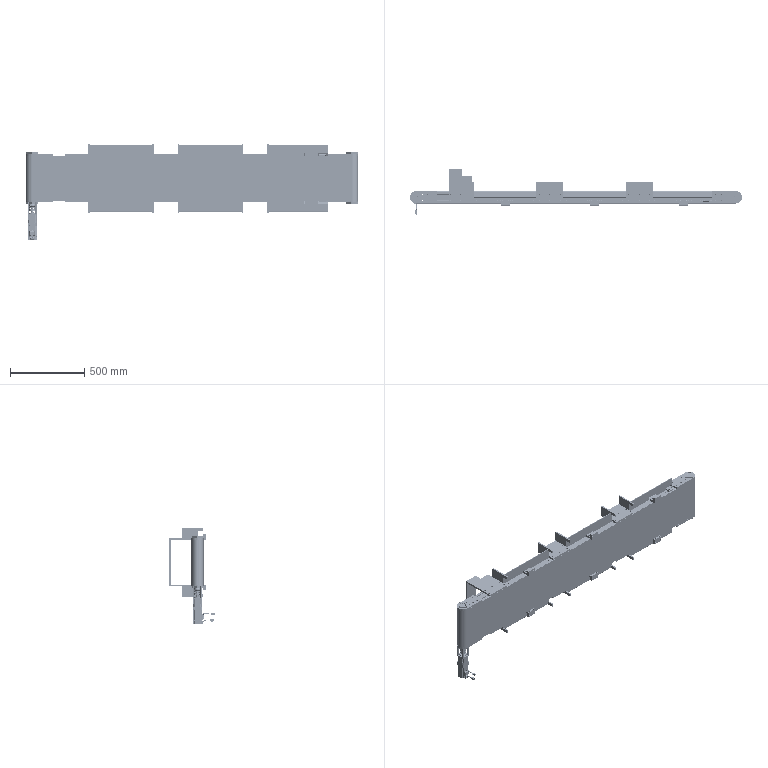Assembly | SolidWorks | mm | 172 component files | 363 solids | 12033 faces | box 2231 x 303.69 x 644.5 mm | volume 22318651 mm3 | plane 6929 | cylinder 3291 | cone 1285 | torus 238 | sphere 160 | spline 130 | commonest cylinder face diameters 8 x392 11 x192 6.6 x192 6 x169 9 x160 13 x160 1 x141 2 x135
Bill of materials:
Q1-A12-S21-Q1A-01A | 2 | S-45C | Flat plate with one rounded end. The rounded end has a large central bore with a ring of small holes around it. The rectangular section has two rows of three holes and two parallel slots on top, and there are notches along the side edges.
Q1-A12-S21-Q1A-02A | 2 | Q235-Steel | Long rectangular bar with two through holes along its length, and chamfers on the two lower long edges.
Q1-A12-S21-Q1A-03A | 1 | SUJ2 | Cylindrical body made of two coaxial larger-diameter sections separated by a narrower neck, with small stepped shaft stubs at both ends.
Q1-CPDW40-16-16 | 1 |  | Cylindrical shaft coupling with two split clamp hubs at the ends and a central spacer ring, joined by thin disc layers held by axial pins or bolts.
Q1-HNTA8-6 | 36 |  | Small block with a trapezoidal top section over a narrower rectangular bottom tongue, giving a stepped profile. It has a single through hole with a chamfered or countersunk entry.
Q1-PAB060-10-S2-P2-14-50-70-Q4 | 1 |  | Square-flanged housing with a round pilot boss and an output shaft on top. Its long body has square edges and longitudinal grooves, and a square base section has a side hole.
Q1-QSQF042L1U2 | 1 |  | Square-flanged, elongated body with a front shaft and a pilot boss. Two side-mounted connector housings have short bent cable leads that end in multi-pin rectangular connector plugs.
Q1-VAFD10-75-F10-Q6-N5 | 4 |  | Long cylindrical pin that steps down at one end to a short smaller-diameter head, with a narrow neck or groove between the head and the main body.
Q1-GNFS8-4080-220 | 6 | 6061 | Extruded profile segment with a rectangular cross-section, roughly 1 x 2 in proportion. It has slots on all sides, a central hollow core and two circular core holes, and a rectangular notch cut partway along the length on both narrow sides.
Q1-HBKTS8-C-SEP | 40 | 6061 | L-shaped angle bracket with a diagonal gusset rib. Each leg carries a socket-head screw that passes through it to a wedge-shaped slot-nut-like piece on the outer face.
Q1-A12-S21-Q1C-01B | 2 | S-45C | Flat plate with one rounded end. The rounded end has a large bore with 4 small holes around it, and the rectangular section has 7 larger holes. Small cross holes or notches appear on one side edge.
Q1-A12-S21-Q1C-02A | 1 | SUJ2 | Cylindrical body made of two coaxial large-diameter sections separated by a narrow neck, with short small-diameter shaft stubs and shoulders at both ends.
Q1-A12-S21-Q1C-03A | 1 | Q235-Steel | Long, slender rectangular bar or thick strip with two small holes drilled into one narrow end face.
Q1-A12-S21-Q1D-01A | 2 | Q235-Steel | Rectangular block with four counterbored through holes in a rectangular pattern, chamfers along two opposite top edges, two raised pads or rails on the underside, and one blind hole in a side face.
Q1-A12-S21-Q4-01A | 4 | SUS-304 | Thin rectangular sheet panel with a joggled (offset) band running across its full width and four small holes near the corners.
Q1-A12-S21-Q4-02A | 6 | SUS-304 | Thin rectangular sheet panel with a joggled offset band across its width and four small corner holes. It looks like the previous panel but is proportionally longer.
Q1-A12-S21-Q4-03A | 4 | White Plastic Steel POM | Thick rectangular plate with six counterbored holes in a 2x3 grid near one edge, three small holes in that edge face, and two short projections on the underside at that edge.
Q1-A12-S21-Q4-05B | 4 | SUS-304 | Bent sheet profile: a horizontal flange with holes, a vertical web, and a hairpin bend at the top that turns into a long angled leg. The flange is split into two tabs by a central notch.
Q1-A12-S21-Q4-06B | 5 | White Plastic Steel POM | Flat L-shaped plate: a rectangular body with a narrow arm sticking out sideways from one top edge, and two small holes near the bottom edge of the body.
Q1-A12-S21-Q4-07B | 1 | SUS-304 | Bent sheet profile with a base flange, a vertical web, a hairpin top bend and an angled leg. The flange is split into one long and one short tab with holes, and the web has rectangular notches in its lower edge between and beyond the tabs.
Q1-A12-S21-Q4-08B | 1 | SUS-304 | Bent sheet profile that looks the same as unnamed part but is shown inverted: a flange with one long and one short tab with holes, a web, a hairpin bend and an angled leg.
Q1-A12-S21-Q4-09B | 5 | White Plastic Steel POM | Flat L-shaped plate with a narrow arm sticking out sideways along one edge and two small holes near the opposite edge. It looks like unnamed part turned over or rotated.
Q1-A12-S21-Q4-10A | 1 | White Plastic Steel POM | Thick plate with a rectangular notch cut from one corner, six counterbored holes in a 2x3 grid near the opposite edge, three small holes in one edge face, and two short projections on the underside.
Q1-A12-S21-Q4-11A | 1 | White Plastic Steel POM | Thick plate with a rectangular notch cut from one corner and six holes in a 2x3 grid. Two narrow raised strips run across the full length of the face shown, and there are three small holes in one edge face. It looks like unnamed part seen from its other side.
Q1-A12-S21-Q4-12A | 1 | White Plastic Steel POM | Thin flat rectangular plate, elongated, with six small through holes: a row of three near each short end.
Q1-A12-S21-Q1E-02A | 6 | Q235-Steel | Rectangular block with two round through holes in its largest face and one chamfer along a single long edge.
Q1-A12-S21-Q4E-01A | 6 | Q235-Steel | Stepped rectangular block: a higher section with two larger through holes, a lower ledge with two smaller through holes, and a narrow rib sticking out of the underside.
Q1-GNFS8-4080-2030 | 2 | 6061 | Long straight extruded bar with a constant slotted cross-section: a rectangle about 2:1 with rounded outer corners, T-shaped slots on all faces, two round core bores, and a central hollow.
Q1-HBLTDS300-4.55 | 1 |  | Long flat bar with fully rounded (semicircular) ends, giving a stadium/obround outline, and a uniform rectangular section through its height.
Mates:
1. coincident | Q1-A12-S21-Q1A.SLDASQ-1/Q1-A12-S21-Q1A-01A-2 face at (48.5, 0, 162.5) dir (0, 0, 1) | Q1-A12-S21-Q1C.SLDASQ-1/Q1-A12-S21-Q1C-01B-1 face at (2089.5, 0, 162.5) dir (0, 0, 1)
2. coincident | Q1-A12-S21-Q1A.SLDASQ-1/Q1-A12-S21-Q1A-01A-2 face at (-41.5, 41.5, 162.5) dir (0, 1, 0) | Q1-A12-S21-Q1C.SLDASQ-1/Q1-A12-S21-Q1C-01B-1 face at (2189.5, 41.5, 162.5) dir (0, 1, 0)
3. distance | Q1-A12-S21-Q1C.SLDASQ-1 plane at (2148, 0, 147.5) dir (-1, 0, 0) | Q1-A12-S21-Q1A.SLDASQ-1 plane at (0, 0, -147.5) dir (1, 0, 0)
4. coincident | Q1-A12-S21-Q1A.SLDASQ-1 plane at (48.5, 0, 0) dir (0, 0, 1) | Q1-HBLTDS300-4.55-1 plane at (0, 0, 0) dir (0, 0, 1)
5. concentric | Q1-A12-S21-Q1A.SLDASQ-1/Q1-A12-S21-Q1A-03A-1 face at (0, 0, -250) dir (0, 0, -1) r 40 | Q1-HBLTDS300-4.55-1 face at (0, 0, -5) dir (0, 0, -1) r 40
6. parallel | Q1-A12-S21-Q1C.SLDASQ-1/Q1-A12-S21-Q1C-01B-1 face at (2189.5, 41.5, 162.5) dir (0, 1, 0) | Q1-HBLTDS300-4.55-1 face at (2148, 41.4, -150) dir (0, 1, 0)
7. coincident | Q1-A12-S21-Q1A.SLDASQ-1/Q1-A12-S21-Q1A-01A-2 face at (-41.5, 41.5, 150) dir (0, 0, -1) | Q1-GNFS8-4080-2030-1 face at (2078.5, 15, 150) dir (0, 0, 1)
8. width | Q1-GNFS8-4080-2030-1 face at (2078.5, 40, 135) dir (0, 1, 0) | Q1-GNFS8-4080-2030-1 face at (2078.5, -40, 147) dir (0, -1, 0) | Q1-A12-S21-Q1A.SLDASQ-1/Q1-A12-S21-Q1A-01A-2 face at (-41.5, -41.5, 162.5) dir (0, -1, 0) | Q1-A12-S21-Q1A.SLDASQ-1/Q1-A12-S21-Q1A-01A-2 face at (-41.5, 41.5, 162.5) dir (0, 1, 0)
9. coincident | Q1-A12-S21-Q1A.SLDASQ-1/Q1-A12-S21-Q1A-02A-2 face at (48.5, -35, 152.5) dir (1, 0, 0) | Q1-GNFS8-4080-2030-1 face at (48.5, 37, 113) dir (-1, 0, 0)
10. coincident | Q1-GNFS8-4080-2030-1 face at (2078.5, 40, 113) dir (0, 1, 0) | Q1-GNFS8-4080-2030-2 face at (2078.5, 40, -147) dir (0, 1, 0)
11. coincident | Q1-A12-S21-Q1A.SLDASQ-1/Q1-A12-S21-Q1A-01A-1 face at (-41.5, -15, -150) dir (0, 0, 1) | Q1-GNFS8-4080-2030-2 face at (2078.5, -15, -150) dir (0, 0, -1)
12. coincident | Q1-A12-S21-Q1A.SLDASQ-1/Q1-A12-S21-Q1A-02A-1 face at (48.5, 35, -152.5) dir (1, 0, 0) | Q1-GNFS8-4080-2030-2 face at (48.5, 37, -147) dir (-1, 0, 0)
13. coincident | Q1-GNFS8-4080-2030-2 face at (2078.5, 40, -125) dir (0, 1, 0) | Q1-GNFS8-4080-220-1 face at (73.5, 40, -110) dir (0, 1, 0)
14. coincident | Q1-GNFS8-4080-2030-2 face at (48.5, 37, -147) dir (-1, 0, 0) | Q1-GNFS8-4080-220-1 face at (48.5, 25, -110) dir (-1, 0, 0)
15. coincident | Q1-GNFS8-4080-2030-2 face at (2078.5, 37, -110) dir (0, 0, 1) | Q1-GNFS8-4080-220-1 face at (51.5, 37, -110) dir (0, 0, -1)
16. coincident | Q1-GNFS8-4080-220-1 face at (73.5, 40, -110) dir (0, 1, 0) | Q1-GNFS8-4080-220-2 face at (2063.5, 40, -110) dir (0, 1, 0)
17. coincident | Q1-GNFS8-4080-2030-1 face at (2078.5, -15, 110) dir (0, 0, -1) | Q1-GNFS8-4080-220-2 face at (2041.5, 37, 110) dir (0, 0, 1)
18. coincident | Q1-GNFS8-4080-2030-2 face at (2078.5, 37, -147) dir (1, 0, 0) | Q1-GNFS8-4080-220-2 face at (2078.5, 15, -110) dir (1, 0, 0)
19. width | Q1-HBKTS8-C-SEP-1 face at (2038.5, 35, -110) dir (0, 1, 0) | Q1-HBKTS8-C-SEP-1 face at (2038.5, 5, -110) dir (0, -1, 0) | Q1-GNFS8-4080-220-2 face at (2038.5, 15, -110) dir (0, 1, 0) | Q1-GNFS8-4080-220-2 face at (2044, 25, -110) dir (0, -1, 0)
20. coincident | Q1-GNFS8-4080-220-2 face at (2038.5, 25, -110) dir (-1, 0, 0) | Q1-HBKTS8-C-SEP-1 face at (2038.5, 35, -59) dir (1, 0, 0)
21. coincident | Q1-GNFS8-4080-2030-2 face at (2078.5, 37, -110) dir (0, 0, 1) | Q1-HBKTS8-C-SEP-1 face at (2038.5, 35, -110) dir (0, 0, -1)
22. width | Q1-HBKTS8-C-SEP-2 face at (2038.5, -5, -110) dir (0, 1, 0) | Q1-HBKTS8-C-SEP-2 face at (2038.5, -35, -110) dir (0, -1, 0) | Q1-GNFS8-4080-220-2 face at (2044, -15, -110) dir (0, -1, 0) | Q1-GNFS8-4080-220-2 face at (2038.5, -25, -110) dir (0, 1, 0)
23. coincident | Q1-GNFS8-4080-220-2 face at (2038.5, -15, -110) dir (-1, 0, 0) | Q1-HBKTS8-C-SEP-2 face at (2038.5, -5, -59) dir (1, 0, 0)
24. coincident | Q1-GNFS8-4080-2030-2 face at (2078.5, 15, -110) dir (0, 0, 1) | Q1-HBKTS8-C-SEP-2 face at (2038.5, -5, -110) dir (0, 0, -1)
25. coincident | Q1-HBKTS8-C-SEP-1 face at (2038.5, 35, -110) dir (0, 1, 0) | Q1-HBKTS8-C-SEP-3 face at (2038.5, 35, 110) dir (0, 1, 0)
26. coincident | Q1-HBKTS8-C-SEP-1 face at (2029.5, 35, -81) dir (-1, 0, 0) | Q1-HBKTS8-C-SEP-3 face at (2029.5, 35, 59) dir (-1, 0, 0)
27. coincident | Q1-GNFS8-4080-2030-1 face at (2078.5, -15, 110) dir (0, 0, -1) | Q1-HBKTS8-C-SEP-3 face at (1987.5, 35, 110) dir (0, 0, 1)
28. coincident | Q1-HBKTS8-C-SEP-2 face at (2038.5, -5, -110) dir (0, 1, 0) | Q1-HBKTS8-C-SEP-4 face at (2038.5, -5, 110) dir (0, 1, 0)
29. coincident | Q1-HBKTS8-C-SEP-3 face at (2029.5, 35, 59) dir (-1, 0, 0) | Q1-HBKTS8-C-SEP-4 face at (2029.5, -5, 59) dir (-1, 0, 0)
30. coincident | Q1-HBKTS8-C-SEP-3 face at (2009.5, 35, 101) dir (0, 0, -1) | Q1-HBKTS8-C-SEP-4 face at (2009.5, -5, 101) dir (0, 0, -1)
31. coincident | Q1-HBKTS8-C-SEP-2 face at (2038.5, -5, -110) dir (0, 1, 0) | Q1-HBKTS8-C-SEP-5 face at (88.5, -5, -110) dir (0, 1, 0)
32. coincident | Q1-GNFS8-4080-2030-2 face at (2078.5, 15, -110) dir (0, 0, 1) | Q1-HBKTS8-C-SEP-5 face at (88.5, -35, -110) dir (0, 0, -1)
33. coincident | Q1-GNFS8-4080-220-1 face at (88.5, 15, -110) dir (1, 0, 0) | Q1-HBKTS8-C-SEP-5 face at (88.5, -35, -59) dir (-1, 0, 0)
34. coincident | Q1-HBKTS8-C-SEP-1 face at (2038.5, 35, -110) dir (0, 1, 0) | Q1-HBKTS8-C-SEP-6 face at (88.5, 35, -110) dir (0, 1, 0)
35. coincident | Q1-GNFS8-4080-2030-2 face at (2078.5, 37, -110) dir (0, 0, 1) | Q1-HBKTS8-C-SEP-6 face at (88.5, 5, -110) dir (0, 0, -1)
36. coincident | Q1-GNFS8-4080-220-1 face at (88.5, 37, -110) dir (1, 0, 0) | Q1-HBKTS8-C-SEP-6 face at (88.5, 5, -59) dir (-1, 0, 0)
37. coincident | Q1-HBKTS8-C-SEP-6 face at (88.5, 35, -110) dir (0, 1, 0) | Q1-HBKTS8-C-SEP-7 face at (88.5, 35, 110) dir (0, 1, 0)
38. coincident | Q1-HBKTS8-C-SEP-6 face at (97.5, 5, -81) dir (1, 0, 0) | Q1-HBKTS8-C-SEP-7 face at (97.5, 5, 59) dir (1, 0, 0)
39. coincident | Q1-GNFS8-4080-2030-1 face at (2078.5, 25, 110) dir (0, 0, -1) | Q1-HBKTS8-C-SEP-7 face at (139.5, 5, 110) dir (0, 0, 1)
40. coincident | Q1-HBKTS8-C-SEP-5 face at (88.5, -5, -110) dir (0, 1, 0) | Q1-HBKTS8-C-SEP-8 face at (88.5, -5, 110) dir (0, 1, 0)
41. coincident | Q1-HBKTS8-C-SEP-7 face at (97.5, 5, 59) dir (1, 0, 0) | Q1-HBKTS8-C-SEP-8 face at (97.5, -35, 59) dir (1, 0, 0)
42. coincident | Q1-HBKTS8-C-SEP-7 face at (117.5, 5, 101) dir (0, 0, -1) | Q1-HBKTS8-C-SEP-8 face at (117.5, -35, 101) dir (0, 0, -1)
43. coincident | Q1-GNFS8-4080-2030-2 face at (2078.5, 40, -125) dir (0, 1, 0) | Q1-A12-S21-Q1B.SLDASQ-1/Q1-GNFS8-4080-220-1 face at (1755.5, 40, 110) dir (0, 1, 0)
44. coincident | Q1-GNFS8-4080-2030-2 face at (2078.5, 37, -110) dir (0, 0, 1) | Q1-A12-S21-Q1B.SLDASQ-1/Q1-GNFS8-4080-220-1 face at (1755.5, 37, -110) dir (0, 0, -1)
45. coincident | Q1-A12-S21-Q1B.SLDASQ-1/Q1-GNFS8-4080-220-1 face at (1733.5, 40, 110) dir (0, 1, 0) | Q1-A12-S21-Q1B.SLDASQ-2/Q1-GNFS8-4080-220-1 face at (1305.5, 40, 110) dir (0, 1, 0)
46. coincident | Q1-GNFS8-4080-2030-2 face at (2078.5, 37, -110) dir (0, 0, 1) | Q1-A12-S21-Q1B.SLDASQ-2/Q1-GNFS8-4080-220-1 face at (1305.5, 37, -110) dir (0, 0, -1)
47. coincident | Q1-GNFS8-4080-2030-2 face at (2078.5, 40, -125) dir (0, 1, 0) | Q1-A12-S21-Q1B.SLDASQ-3/Q1-GNFS8-4080-220-1 face at (855.5, 40, 110) dir (0, 1, 0)
48. coincident | Q1-GNFS8-4080-2030-2 face at (2078.5, 37, -110) dir (0, 0, 1) | Q1-A12-S21-Q1B.SLDASQ-3/Q1-GNFS8-4080-220-1 face at (855.5, 37, -110) dir (0, 0, -1)
49. coincident | Q1-GNFS8-4080-2030-2 face at (2078.5, 40, -125) dir (0, 1, 0) | Q1-A12-S21-Q1B.SLDASQ-4/Q1-GNFS8-4080-220-1 face at (405.5, 40, 110) dir (0, 1, 0)
50. coincident | Q1-GNFS8-4080-2030-2 face at (2078.5, 15, -110) dir (0, 0, 1) | Q1-A12-S21-Q1B.SLDASQ-4/Q1-GNFS8-4080-220-1 face at (405.5, 37, -110) dir (0, 0, -1)
51. distance | Q1-GNFS8-4080-220-1 face at (48.5, 25, -110) dir (-1, 0, 0) | Q1-A12-S21-Q1B.SLDASQ-4/Q1-GNFS8-4080-220-1 face at (368.5, 37, 110) dir (-1, 0, 0)
52. distance | Q1-A12-S21-Q1B.SLDASQ-2/Q1-GNFS8-4080-220-1 face at (1268.5, 37, 110) dir (-1, 0, 0) | Q1-A12-S21-Q1B.SLDASQ-3/Q1-GNFS8-4080-220-1 face at (858.5, 25, 110) dir (1, 0, 0)
53. distance | Q1-A12-S21-Q1B.SLDASQ-1/Q1-GNFS8-4080-220-1 face at (1718.5, 37, 110) dir (-1, 0, 0) | Q1-A12-S21-Q1B.SLDASQ-2/Q1-GNFS8-4080-220-1 face at (1308.5, 25, 110) dir (1, 0, 0)
54. distance | Q1-A12-S21-Q1B.SLDASQ-3/Q1-GNFS8-4080-220-1 face at (818.5, 37, 110) dir (-1, 0, 0) | Q1-A12-S21-Q1B.SLDASQ-4/Q1-GNFS8-4080-220-1 face at (408.5, 25, 110) dir (1, 0, 0)
55. width | Q1-A12-S21-Q1D.SLDASQ-1/Q1-A12-S21-Q1D-01A-1 face at (1929.5, 30, 162.5) dir (0, 1, 0) | Q1-A12-S21-Q1D.SLDASQ-1/Q1-A12-S21-Q1D-01A-1 face at (1929.5, -30, 162.5) dir (0, -1, 0) | Q1-A12-S21-Q1C.SLDASQ-1/Q1-A12-S21-Q1C-01B-1 face at (2189.5, -41.5, 162.5) dir (0, -1, 0) | Q1-A12-S21-Q1C.SLDASQ-1/Q1-A12-S21-Q1C-01B-1 face at (2189.5, 41.5, 162.5) dir (0, 1, 0)
56. coincident | Q1-GNFS8-4080-2030-1 face at (2078.5, 37, 150) dir (0, 0, 1) | Q1-A12-S21-Q1D.SLDASQ-1/Q1-A12-S21-Q1D-01A-1 face at (1929.5, 30, 150) dir (0, 0, -1)
57. coincident | Q1-A12-S21-Q1C.SLDASQ-1/Q1-A12-S21-Q1C-01B-1 face at (1989.5, 41.5, 162.5) dir (-1, 0, 0) | Q1-A12-S21-Q1D.SLDASQ-1/Q1-RCB6-30-1 face at (1989.5, 0, 156.25) dir (1, 0, 0)
58. coincident | Q1-GNFS8-4080-2030-2 face at (2078.5, 25, -150) dir (0, 0, -1) | Q1-A12-S21-Q1D.SLDASQ-2/Q1-A12-S21-Q1D-01A-1 face at (1929.5, 30, -150) dir (0, 0, 1)
59. width | Q1-A12-S21-Q1C.SLDASQ-1/Q1-A12-S21-Q1C-01B-2 face at (2189.5, 41.5, -162.5) dir (0, 1, 0) | Q1-A12-S21-Q1C.SLDASQ-1/Q1-A12-S21-Q1C-01B-2 face at (2189.5, -41.5, -162.5) dir (0, -1, 0) | Q1-A12-S21-Q1D.SLDASQ-2/Q1-A12-S21-Q1D-01A-1 face at (1929.5, -30, -162.5) dir (0, -1, 0) | Q1-A12-S21-Q1D.SLDASQ-2/Q1-A12-S21-Q1D-01A-1 face at (1929.5, 30, -162.5) dir (0, 1, 0)
60. coincident | Q1-A12-S21-Q1C.SLDASQ-1/Q1-A12-S21-Q1C-01B-2 face at (1989.5, -41.5, -162.5) dir (-1, 0, 0) | Q1-A12-S21-Q1D.SLDASQ-2/Q1-RCB6-30-1 face at (1989.5, 0, -156.25) dir (1, 0, 0)
61. coincident | Q1-HBKTS8-C-SEP-3 face at (2038.5, 35, 110) dir (0, 1, 0) | Q1-A12-S21-Q4-01A-1 face at (1898.5, 35, -71.578) dir (0, -1, 0)
62. concentric | Q1-HBKTS8-C-SEP-1 face at (2026.5, 5, -98) dir (0, 1, 0) r 2.067 | Q1-A12-S21-Q4-01A-1 face at (2026.5, 39, -98) dir (0, 1, 0) r 2.75
63. parallel | Q1-GNFS8-4080-220-2 face at (2038.5, 25, -110) dir (-1, 0, 0) | Q1-A12-S21-Q4-01A-1 face at (2038.5, 39, 25.053) dir (1, 0, 0)
64. coincident | Q1-HBKTS8-C-SEP-7 face at (88.5, 35, 110) dir (0, 1, 0) | Q1-A12-S21-Q4-01A-2 face at (228.5, 35, -71.578) dir (0, -1, 0)
65. concentric | Q1-HBKTS8-C-SEP-6 face at (100.5, 35, -98) dir (0, -1, 0) r 2.067 | Q1-A12-S21-Q4-01A-2 face at (100.5, 39, -98) dir (0, 1, 0) r 2.75
66. parallel | Q1-GNFS8-4080-220-1 face at (88.5, 37, -110) dir (1, 0, 0) | Q1-A12-S21-Q4-01A-2 face at (88.5, 39, 110) dir (-1, 0, 0)
67. coincident | Q1-A12-S21-Q1B.SLDASQ-3/Q1-HBKTS8-C-SEP-7 face at (818.5, 35, -110) dir (0, 1, 0) | Q1-A12-S21-Q4-02A-1 face at (613.5, 35, -63) dir (0, -1, 0)
68. concentric | Q1-A12-S21-Q1B.SLDASQ-3/Q1-HBKTS8-C-SEP-7 face at (806.5, 5, -98) dir (0, 1, 0) r 2.067 | Q1-A12-S21-Q4-02A-1 face at (806.5, 39, -98) dir (0, 1, 0) r 2.75
69. parallel | Q1-A12-S21-Q1B.SLDASQ-3/Q1-GNFS8-4080-220-1 face at (818.5, 37, 110) dir (-1, 0, 0) | Q1-A12-S21-Q4-02A-1 face at (818.5, 39, 25.053) dir (1, 0, 0)
70. coincident | Q1-A12-S21-Q1B.SLDASQ-2/Q1-HBKTS8-C-SEP-7 face at (1268.5, 35, -110) dir (0, 1, 0) | Q1-A12-S21-Q4-02A-2 face at (1063.5, 35, -63) dir (0, -1, 0)
71. concentric | Q1-A12-S21-Q1B.SLDASQ-2/Q1-HBKTS8-C-SEP-7 face at (1256.5, 5, -98) dir (0, 1, 0) r 2.067 | Q1-A12-S21-Q4-02A-2 face at (1256.5, 39, -98) dir (0, 1, 0) r 2.75
72. parallel | Q1-A12-S21-Q1B.SLDASQ-2/Q1-GNFS8-4080-220-1 face at (1268.5, 37, 110) dir (-1, 0, 0) | Q1-A12-S21-Q4-02A-2 face at (1268.5, 39, 25.053) dir (1, 0, 0)
73. coincident | Q1-A12-S21-Q1B.SLDASQ-1/Q1-HBKTS8-C-SEP-7 face at (1718.5, 35, -110) dir (0, 1, 0) | Q1-A12-S21-Q4-02A-3 face at (1513.5, 35, -63) dir (0, -1, 0)
74. concentric | Q1-A12-S21-Q1B.SLDASQ-1/Q1-HBKTS8-C-SEP-7 face at (1706.5, 5, -98) dir (0, 1, 0) r 2.067 | Q1-A12-S21-Q4-02A-3 face at (1706.5, 39, -98) dir (0, 1, 0) r 2.75
75. parallel | Q1-A12-S21-Q1B.SLDASQ-1/Q1-GNFS8-4080-220-1 face at (1718.5, 37, 110) dir (-1, 0, 0) | Q1-A12-S21-Q4-02A-3 face at (1718.5, 39, 25.053) dir (1, 0, 0)
76. coincident | Q1-HBKTS8-C-SEP-4 face at (2038.5, -35, 110) dir (0, -1, 0) | Q1-A12-S21-Q4-01A-3 face at (1898.5, -35, 63) dir (0, 1, 0)
77. concentric | Q1-HBKTS8-C-SEP-4 face at (2026.5, -35, 98) dir (0, 1, 0) r 2.067 | Q1-A12-S21-Q4-01A-3 face at (2026.5, -39, 98) dir (0, -1, 0) r 2.75
78. parallel | Q1-GNFS8-4080-220-2 face at (2038.5, -37, -110) dir (-1, 0, 0) | Q1-A12-S21-Q4-01A-3 face at (2038.5, -35, 16) dir (1, 0, 0)
79. coincident | Q1-A12-S21-Q1B.SLDASQ-1/Q1-HBKTS8-C-SEP-6 face at (1718.5, -35, 110) dir (0, -1, 0) | Q1-A12-S21-Q4-02A-4 face at (1513.5, -35, 63) dir (0, 1, 0)
80. concentric | Q1-A12-S21-Q1B.SLDASQ-1/Q1-HBKTS8-C-SEP-6 face at (1706.5, -35, 98) dir (0, 1, 0) r 2.067 | Q1-A12-S21-Q4-02A-4 face at (1706.5, -39, 98) dir (0, -1, 0) r 2.75
81. parallel | Q1-A12-S21-Q1B.SLDASQ-1/Q1-GNFS8-4080-220-1 face at (1718.5, -25, 110) dir (-1, 0, 0) | Q1-A12-S21-Q4-02A-4 face at (1718.5, -35, 16) dir (1, 0, 0)
82. coincident | Q1-A12-S21-Q1B.SLDASQ-2/Q1-HBKTS8-C-SEP-6 face at (1268.5, -35, 110) dir (0, -1, 0) | Q1-A12-S21-Q4-02A-5 face at (1063.5, -35, 63) dir (0, 1, 0)
83. concentric | Q1-A12-S21-Q1B.SLDASQ-2/Q1-HBKTS8-C-SEP-6 face at (1256.5, -35, 98) dir (0, 1, 0) r 2.067 | Q1-A12-S21-Q4-02A-5 face at (1256.5, -39, 98) dir (0, -1, 0) r 2.75
84. parallel | Q1-A12-S21-Q1B.SLDASQ-2/Q1-GNFS8-4080-220-1 face at (1268.5, -25, 110) dir (-1, 0, 0) | Q1-A12-S21-Q4-02A-5 face at (1268.5, -35, 16) dir (1, 0, 0)
85. coincident | Q1-A12-S21-Q1B.SLDASQ-3/Q1-HBKTS8-C-SEP-6 face at (818.5, -35, 110) dir (0, -1, 0) | Q1-A12-S21-Q4-02A-6 face at (613.5, -35, 63) dir (0, 1, 0)
86. concentric | Q1-A12-S21-Q1B.SLDASQ-3/Q1-HBKTS8-C-SEP-6 face at (806.5, -35, 98) dir (0, 1, 0) r 2.067 | Q1-A12-S21-Q4-02A-6 face at (806.5, -39, 98) dir (0, -1, 0) r 2.75
87. parallel | Q1-A12-S21-Q1B.SLDASQ-3/Q1-GNFS8-4080-220-1 face at (818.5, -25, 110) dir (-1, 0, 0) | Q1-A12-S21-Q4-02A-6 face at (818.5, -35, 16) dir (1, 0, 0)
88. coincident | Q1-A12-S21-Q1B.SLDASQ-4/Q1-HBKTS8-C-SEP-6 face at (368.5, -35, 110) dir (0, -1, 0) | Q1-A12-S21-Q4-01A-4 face at (228.5, -35, 63) dir (0, 1, 0)
89. concentric | Q1-A12-S21-Q1B.SLDASQ-4/Q1-HBKTS8-C-SEP-6 face at (356.5, -35, 98) dir (0, 1, 0) r 2.067 | Q1-A12-S21-Q4-01A-4 face at (356.5, -39, 98) dir (0, -1, 0) r 2.75
90. parallel | Q1-A12-S21-Q1B.SLDASQ-4/Q1-GNFS8-4080-220-1 face at (368.5, -25, 110) dir (-1, 0, 0) | Q1-A12-S21-Q4-01A-4 face at (368.5, -35, 16) dir (1, 0, 0)
91. coincident | Q1-GNFS8-4080-2030-1 face at (2078.5, 15, 150) dir (0, 0, 1) | Q1-A12-S21-Q4E.SLDASQ-4/Q1-A12-S21-Q4E-01A-1 face at (1768.5, -5, 150) dir (0, 0, -1)
92. distance | Q1-GNFS8-4080-2030-1 face at (2078.5, 37, 113) dir (1, 0, 0) | Q1-A12-S21-Q4E.SLDASQ-4/Q1-A12-S21-Q4E-01A-1 face at (1828.5, -55, 165) dir (1, 0, 0)
93. coincident | Q1-A12-S21-Q4E.SLDASQ-4/Q1-A12-S21-Q1E-02A-1 face at (1798.5, -40, 174) dir (0, 1, 0) | Q1-A12-S21-Q4E.SLDASQ-5/Q1-A12-S21-Q1E-02A-1 face at (1198.5, -40, 174) dir (0, 1, 0)
94. coincident | Q1-A12-S21-Q4E.SLDASQ-4/Q1-A12-S21-Q4E-01A-1 face at (1798.5, -30, 165) dir (0, 0, 1) | Q1-A12-S21-Q4E.SLDASQ-5/Q1-A12-S21-Q4E-01A-1 face at (1198.5, -30, 165) dir (0, 0, 1)
95. coincident | Q1-A12-S21-Q4E.SLDASQ-5/Q1-A12-S21-Q4E-01A-1 face at (1198.5, -30, 165) dir (0, 0, 1) | Q1-A12-S21-Q4E.SLDASQ-6/Q1-A12-S21-Q4E-01A-1 face at (598.5, -30, 165) dir (0, 0, 1)
96. coincident | Q1-A12-S21-Q4E.SLDASQ-5/Q1-A12-S21-Q1E-02A-1 face at (1198.5, -40, 174) dir (0, 1, 0) | Q1-A12-S21-Q4E.SLDASQ-6/Q1-A12-S21-Q1E-02A-1 face at (598.5, -40, 174) dir (0, 1, 0)
97. coincident | Q1-GNFS8-4080-2030-2 face at (2078.5, -15, -150) dir (0, 0, -1) | Q1-A12-S21-Q4E.SLDASQ-7/Q1-A12-S21-Q4E-01A-1 face at (1828.5, -5, -150) dir (0, 0, 1)
98. coincident | Q1-A12-S21-Q4E.SLDASQ-4/Q1-A12-S21-Q1E-02A-1 face at (1798.5, -40, 174) dir (0, 1, 0) | Q1-A12-S21-Q4E.SLDASQ-7/Q1-A12-S21-Q1E-02A-1 face at (1798.5, -40, -174) dir (0, 1, 0)
99. coincident | Q1-A12-S21-Q4E.SLDASQ-4/Q1-A12-S21-Q4E-01A-1 face at (1828.5, -55, 165) dir (1, 0, 0) | Q1-A12-S21-Q4E.SLDASQ-7/Q1-A12-S21-Q4E-01A-1 face at (1828.5, -55, -165) dir (1, 0, 0)
100. coincident | Q1-A12-S21-Q4E.SLDASQ-7/Q1-A12-S21-Q4E-01A-1 face at (1798.5, -30, -165) dir (0, 0, -1) | Q1-A12-S21-Q4E.SLDASQ-8/Q1-A12-S21-Q4E-01A-1 face at (1198.5, -30, -165) dir (0, 0, -1)
101. coincident | Q1-A12-S21-Q4E.SLDASQ-7/Q1-A12-S21-Q1E-02A-1 face at (1798.5, -40, -174) dir (0, 1, 0) | Q1-A12-S21-Q4E.SLDASQ-8/Q1-A12-S21-Q1E-02A-1 face at (1198.5, -40, -174) dir (0, 1, 0)
102. coincident | Q1-A12-S21-Q4E.SLDASQ-5/Q1-A12-S21-Q4E-01A-1 face at (1228.5, -55, 165) dir (1, 0, 0) | Q1-A12-S21-Q4E.SLDASQ-8/Q1-A12-S21-Q4E-01A-1 face at (1228.5, -55, -165) dir (1, 0, 0)
103. coincident | Q1-A12-S21-Q4E.SLDASQ-8/Q1-A12-S21-Q4E-01A-1 face at (1198.5, -30, -165) dir (0, 0, -1) | Q1-A12-S21-Q4E.SLDASQ-9/Q1-A12-S21-Q4E-01A-1 face at (598.5, -30, -165) dir (0, 0, -1)
104. coincident | Q1-A12-S21-Q4E.SLDASQ-8/Q1-A12-S21-Q1E-02A-1 face at (1198.5, -40, -174) dir (0, 1, 0) | Q1-A12-S21-Q4E.SLDASQ-9/Q1-A12-S21-Q1E-02A-1 face at (598.5, -40, -174) dir (0, 1, 0)
105. coincident | Q1-A12-S21-Q4E.SLDASQ-6/Q1-A12-S21-Q4E-01A-1 face at (628.5, -55, 165) dir (1, 0, 0) | Q1-A12-S21-Q4E.SLDASQ-9/Q1-A12-S21-Q4E-01A-1 face at (628.5, -55, -165) dir (1, 0, 0)
106. coincident | Q1-GNFS8-4080-2030-1 face at (2078.5, -25, 150) dir (0, 0, 1) | Q1-A12-S21-Q4-10A-1 face at (218.5, -15.9, 150) dir (0, 0, -1)
107. coincident | Q1-GNFS8-4080-2030-1 face at (2078.5, -40, 147) dir (0, -1, 0) | Q1-A12-S21-Q4-10A-1 face at (218.5, -40, 162.5) dir (0, -1, 0)
108. coincident | Q1-GNFS8-4080-2030-1 face at (2078.5, -25, 150) dir (0, 0, 1) | Q1-A12-S21-Q4-05B-1 face at (598.5, -20, 150) dir (0, 0, -1)
109. coincident | Q1-GNFS8-4080-2030-1 face at (2078.5, -40, 147) dir (0, -1, 0) | Q1-A12-S21-Q4-05B-1 face at (388.5, -40, 150) dir (0, -1, 0)
110. distance | Q1-A12-S21-Q4-10A-1 face at (378.5, -40, 162.5) dir (1, 0, 0) | Q1-A12-S21-Q4-05B-1 face at (388.5, 0, 230) dir (-1, 0, 0)
111. width | Q1-A12-S21-Q4E.SLDASQ-4/Q1-A12-S21-Q4E-01A-1 face at (1768.5, -15, 147.5) dir (0, 1, 0) | Q1-A12-S21-Q4E.SLDASQ-4/Q1-A12-S21-Q4E-01A-1 face at (1768.5, -25, 147.5) dir (0, -1, 0) | Q1-GNFS8-4080-2030-1 face at (2078.5, -15, 150) dir (0, -1, 0) | Q1-GNFS8-4080-2030-1 face at (2078.5, -25, 144.5) dir (0, 1, 0)
112. coincident | Q1-A12-S21-Q4-10A-1 face at (378.5, -40, 162.5) dir (1, 0, 0) | Q1-A12-S21-Q4-06B-1 face at (378.5, 30, 190) dir (-1, 0, 0)
113. coincident | Q1-A12-S21-Q4-10A-1 face at (218.5, -40, 162.5) dir (0, -1, 0) | Q1-A12-S21-Q4-06B-1 face at (388.5, -40, 230) dir (0, -1, 0)
114. coincident | Q1-A12-S21-Q4-10A-1 face at (218.5, 24.1, 150) dir (0, 0, -1) | Q1-A12-S21-Q4-06B-1 face at (388.5, -40, 150) dir (0, 0, -1)
115. coincident | Q1-A12-S21-Q4-10A-1 face at (298.5, 70, 162.5) dir (0, 0, 1) | Q1-A12-S21-Q4-03A-2 face at (898.5, 30, 162.5) dir (0, 0, 1)
116. coincident | Q1-A12-S21-Q4-10A-1 face at (218.5, -40, 162.5) dir (0, -1, 0) | Q1-A12-S21-Q4-03A-2 face at (818.5, -40, 162.5) dir (0, -1, 0)
117. concentric | Q1-A12-S21-Q4-03A-2 face at (818.5, 70, 157) dir (-1, 0, 0) r 1.65 | Q1-A12-S21-Q4-09B-5 face at (808.5, 70, 157) dir (-1, 0, 0) r 4
118. coincident | Q1-A12-S21-Q4-05B-1 face at (598.5, -20, 151.5) dir (0, 0, 1) | Q1-A12-S21-Q4-07B-1 face at (1788.5, -20, 151.5) dir (0, 0, 1)
119. coincident | Q1-A12-S21-Q4-05B-1 face at (388.5, -40, 150) dir (0, -1, 0) | Q1-A12-S21-Q4-07B-1 face at (1588.5, -40, 150) dir (0, -1, 0)
120. coincident | Q1-A12-S21-Q4-03A-2 face at (978.5, -40, 162.5) dir (1, 0, 0) | Q1-A12-S21-Q4-06B-9 face at (978.5, 30, 190) dir (-1, 0, 0)
121. coincident | Q1-A12-S21-Q4-09B-5 face at (808.5, -40, 230) dir (0, -1, 0) | Q1-A12-S21-Q4-06B-9 face at (988.5, -40, 230) dir (0, -1, 0)
122. coincident | Q1-A12-S21-Q4-09B-5 face at (808.5, 100, 230) dir (0, 0, 1) | Q1-A12-S21-Q4-06B-9 face at (988.5, -40, 230) dir (0, 0, 1)
123. coincident | Q1-A12-S21-Q4-03A-2 face at (898.5, 30, 162.5) dir (0, 0, 1) | Q1-A12-S21-Q4-03A-7 face at (1498.5, 30, 162.5) dir (0, 0, 1)
124. coincident | Q1-A12-S21-Q4-03A-2 face at (818.5, -40, 162.5) dir (0, -1, 0) | Q1-A12-S21-Q4-03A-7 face at (1418.5, -40, 162.5) dir (0, -1, 0)
125. coincident | Q1-A12-S21-Q4-03A-7 face at (1418.5, -40, 162.5) dir (-1, 0, 0) | Q1-A12-S21-Q4-09B-6 face at (1418.5, 30, 190) dir (1, 0, 0)
126. concentric | Q1-A12-S21-Q4-03A-7 face at (1418.5, 70, 157) dir (-1, 0, 0) r 1.65 | Q1-A12-S21-Q4-09B-6 face at (1408.5, 70, 157) dir (-1, 0, 0) r 4
127. coincident | Q1-A12-S21-Q4-03A-7 face at (1578.5, -40, 162.5) dir (1, 0, 0) | Q1-A12-S21-Q4-06B-5 face at (1578.5, 30, 190) dir (-1, 0, 0)
128. concentric | Q1-A12-S21-Q4-03A-7 face at (1578.5, 70, 157) dir (1, 0, 0) r 1.65 | Q1-A12-S21-Q4-06B-5 face at (1588.5, 70, 157) dir (1, 0, 0) r 4
129. coincident | Q1-A12-S21-Q4-10A-1 face at (218.5, -40, 162.5) dir (-1, 0, 0) | Q1-A12-S21-Q4-11A-4 face at (218.5, -40, -162.5) dir (-1, 0, 0)
130. coincident | Q1-A12-S21-Q4-10A-1 face at (218.5, -40, 162.5) dir (0, -1, 0) | Q1-A12-S21-Q4-11A-4 face at (378.5, -40, -162.5) dir (0, -1, 0)
131. coincident | Q1-GNFS8-4080-2030-2 face at (2078.5, -37, -150) dir (0, 0, -1) | Q1-A12-S21-Q4-11A-4 face at (378.5, 24.1, -150) dir (0, 0, 1)
132. concentric | Q1-A12-S21-Q4-11A-4 face at (378.5, 70, -157) dir (1, 0, 0) r 1.65 | Q1-A12-S21-Q4-09B-7 face at (388.5, 70, -157) dir (1, 0, 0) r 4
133. coincident | Q1-A12-S21-Q4-11A-4 face at (378.5, -40, -162.5) dir (1, 0, 0) | Q1-A12-S21-Q4-09B-7 face at (378.5, 30, -190) dir (-1, 0, 0)
134. distance | Q1-A12-S21-Q4E.SLDASQ-5 plane at (1198.5, -30, 147.5) dir (1, 0, 0) | Q1-A12-S21-Q4E.SLDASQ-4 plane at (1798.5, -30, 147.5) dir (1, 0, 0)
135. distance | Q1-A12-S21-Q4E.SLDASQ-6 plane at (598.5, -30, 147.5) dir (1, 0, 0) | Q1-A12-S21-Q4E.SLDASQ-5 plane at (1198.5, -30, 147.5) dir (1, 0, 0)
136. distance | Q1-A12-S21-Q4-10A-1 face at (218.5, -40, 162.5) dir (-1, 0, 0) | Q1-A12-S21-Q1A.SLDASQ-1/Q1-A12-S21-Q1A-01A-2 face at (138.5, -41.5, 162.5) dir (1, 0, 0)
137. coincident | Q1-A12-S21-Q4-07B-1 face at (1588.5, 0, 230) dir (-1, 0, 0) | Q1-A12-S21-Q4-06B-5 face at (1588.5, 30, 190) dir (1, 0, 0)
138. coincident | Q1-A12-S21-Q4-05B-1 face at (388.5, -40, 150) dir (0, -1, 0) | Q1-A12-S21-Q4-05B-2 edge at (988.5, -40, 151.5) dir (1, 0, 0)
139. coincident | Q1-A12-S21-Q4-05B-1 face at (598.5, -20, 151.5) dir (0, 0, 1) | Q1-A12-S21-Q4-05B-2 face at (1198.5, -20, 151.5) dir (0, 0, 1)
140. coincident | Q1-A12-S21-Q4-06B-9 face at (988.5, 30, 190) dir (1, 0, 0) | Q1-A12-S21-Q4-05B-2 face at (988.5, 0, 230) dir (-1, 0, 0)
141. coincident | Q1-A12-S21-Q4-09B-6 face at (1408.5, 30, 190) dir (-1, 0, 0) | Q1-A12-S21-Q4-05B-2 edge at (1408.5, 0, 223.128) dir (0, 0, -1)
142. coincident | Q1-A12-S21-Q4-05B-1 face at (388.5, -40, 150) dir (0, -1, 0) | Q1-A12-S21-Q4-05B-3 face at (808.5, -40, -150) dir (0, -1, 0)
143. coincident | Q1-GNFS8-4080-2030-2 face at (2078.5, -15, -150) dir (0, 0, -1) | Q1-A12-S21-Q4-05B-3 face at (598.5, -20, -150) dir (0, 0, 1)
144. coincident | Q1-A12-S21-Q4-09B-7 face at (388.5, 30, -190) dir (1, 0, 0) | Q1-A12-S21-Q4-05B-3 face at (388.5, -40, -150) dir (-1, 0, 0)
145. coincident | Q1-A12-S21-Q4-11A-4 face at (298.5, 70, -162.5) dir (0, 0, -1) | Q1-A12-S21-Q4-03A-5 face at (898.5, 30, -162.5) dir (0, 0, -1)
146. coincident | Q1-A12-S21-Q4-03A-5 face at (898.5, 30, -162.5) dir (0, 0, -1) | Q1-A12-S21-Q4-03A-6 face at (1498.5, 30, -162.5) dir (0, 0, -1)
147. coincident | Q1-A12-S21-Q4-03A-5 face at (978.5, 100, -162.5) dir (0, 1, 0) | Q1-A12-S21-Q4-03A-6 face at (1578.5, 100, -162.5) dir (0, 1, 0)
148. concentric | Q1-A12-S21-Q4-06B-7 face at (808.5, 70, -157) dir (-1, 0, 0) r 4 | Q1-A12-S21-Q4-03A-5 face at (818.5, 70, -157) dir (-1, 0, 0) r 1.65
149. coincident | Q1-A12-S21-Q4-06B-7 face at (818.5, 30, -190) dir (1, 0, 0) | Q1-A12-S21-Q4-03A-5 face at (818.5, -40, -162.5) dir (-1, 0, 0)
150. concentric | Q1-A12-S21-Q4-03A-6 face at (1418.5, 70, -157) dir (-1, 0, 0) r 1.65 | Q1-A12-S21-Q4-06B-8 face at (1408.5, 70, -157) dir (-1, 0, 0) r 4
151. coincident | Q1-A12-S21-Q4-03A-6 face at (1418.5, -40, -162.5) dir (-1, 0, 0) | Q1-A12-S21-Q4-06B-8 face at (1418.5, 30, -190) dir (1, 0, 0)
152. coincident | Q1-A12-S21-Q4-03A-5 face at (978.5, -40, -162.5) dir (1, 0, 0) | Q1-A12-S21-Q4-09B-9 face at (978.5, 30, -190) dir (-1, 0, 0)
153. concentric | Q1-A12-S21-Q4-03A-5 face at (978.5, 70, -157) dir (1, 0, 0) r 1.65 | Q1-A12-S21-Q4-09B-9 face at (988.5, 70, -157) dir (1, 0, 0) r 4
154. coincident | Q1-A12-S21-Q4-03A-6 face at (1578.5, -40, -162.5) dir (1, 0, 0) | Q1-A12-S21-Q4-09B-10 face at (1578.5, 30, -190) dir (-1, 0, 0)
155. concentric | Q1-A12-S21-Q4-03A-6 face at (1578.5, 70, -157) dir (1, 0, 0) r 1.65 | Q1-A12-S21-Q4-09B-10 face at (1588.5, 70, -157) dir (1, 0, 0) r 4
156. coincident | Q1-A12-S21-Q4-05B-3 face at (808.5, 0, -230) dir (1, 0, 0) | Q1-A12-S21-Q4-06B-7 face at (808.5, 30, -190) dir (-1, 0, 0)
157. coincident | Q1-A12-S21-Q4-05B-3 face at (598.5, -20, -151.5) dir (0, 0, -1) | Q1-A12-S21-Q4-05B-4 face at (1198.5, -20, -151.5) dir (0, 0, -1)
158. coincident | Q1-A12-S21-Q4-05B-3 face at (808.5, -40, -150) dir (0, -1, 0) | Q1-A12-S21-Q4-05B-4 face at (1408.5, -40, -150) dir (0, -1, 0)
159. coincident | Q1-A12-S21-Q4-09B-9 face at (988.5, 30, -190) dir (1, 0, 0) | Q1-A12-S21-Q4-05B-4 face at (988.5, 0, -151.5) dir (-1, 0, 0)
160. coincident | Q1-A12-S21-Q4-06B-8 face at (1408.5, 30, -190) dir (-1, 0, 0) | Q1-A12-S21-Q4-05B-4 face at (1408.5, 0, -230) dir (1, 0, 0)
161. coincident | Q1-A12-S21-Q4-05B-4 face at (1198.5, -20, -151.5) dir (0, 0, -1) | Q1-A12-S21-Q4-08B-2 face at (1788.5, -20, -151.5) dir (0, 0, -1)
162. coincident | Q1-A12-S21-Q4-05B-4 face at (1408.5, -40, -150) dir (0, -1, 0) | Q1-A12-S21-Q4-08B-2 face at (1988.5, -40, -150) dir (0, -1, 0)
163. coincident | Q1-A12-S21-Q4-09B-10 face at (1588.5, 30, -190) dir (1, 0, 0) | Q1-A12-S21-Q4-08B-2 face at (1588.5, -40, -150) dir (-1, 0, 0)
164. concentric | Q1-A12-S21-Q4-03A-7 face at (1418.5, 30, 157) dir (-1, 0, 0) r 1.65 | Q1-A12-S21-Q4-09B-6 face at (1408.5, 30, 157) dir (-1, 0, 0) r 2.25
165. concentric | Q1-A12-S21-Q4-03A-2 face at (818.5, 30, 157) dir (-1, 0, 0) r 1.65 | Q1-A12-S21-Q4-09B-5 face at (808.5, 30, 157) dir (-1, 0, 0) r 4
166. coincident | Q1-A12-S21-Q4-03A-2 face at (818.5, -40, 162.5) dir (-1, 0, 0) | Q1-A12-S21-Q4-09B-5 face at (818.5, 30, 190) dir (1, 0, 0)
167. distance | Q1-A12-S21-Q4-09B-5 face at (808.5, 30, 190) dir (-1, 0, 0) | Q1-A12-S21-Q1A.SLDASQ-1/Q1-A12-S21-Q1A-01A-2 face at (138.5, -41.5, 162.5) dir (1, 0, 0)
168. concentric | Q1-A12-S21-Q4-11A-4 face at (378.5, 30, -157) dir (1, 0, 0) r 1.65 | Q1-A12-S21-Q4-09B-7 face at (388.5, 30, -157) dir (1, 0, 0) r 4
169. concentric | Q1-A12-S21-Q4-03A-5 face at (978.5, 30, -157) dir (1, 0, 0) r 1.65 | Q1-A12-S21-Q4-09B-9 face at (988.5, 30, -157) dir (1, 0, 0) r 4
170. concentric | Q1-A12-S21-Q4-03A-6 face at (1578.5, 30, -157) dir (1, 0, 0) r 1.65 | Q1-A12-S21-Q4-09B-10 face at (1588.5, 30, -157) dir (1, 0, 0) r 4
171. concentric | Q1-A12-S21-Q4-06B-7 face at (808.5, 30, -157) dir (-1, 0, 0) r 4 | Q1-A12-S21-Q4-03A-5 face at (818.5, 30, -157) dir (-1, 0, 0) r 1.65
172. concentric | Q1-A12-S21-Q4-03A-6 face at (1418.5, 30, -157) dir (-1, 0, 0) r 1.65 | Q1-A12-S21-Q4-06B-8 face at (1408.5, 30, -157) dir (-1, 0, 0) r 4
173. concentric | Q1-A12-S21-Q4-03A-7 face at (1578.5, 30, 157) dir (1, 0, 0) r 1.65 | Q1-A12-S21-Q4-06B-5 face at (1588.5, 30, 157) dir (1, 0, 0) r 4
174. coincident | Q1-GNFS8-4080-2030-2 face at (2078.5, -40, -135) dir (0, -1, 0) | Q1-A12-S21-Q4-03A-5 face at (978.5, -40, -162.5) dir (0, -1, 0)
175. coincident | Q1-A12-S21-Q4-10A-1 face at (218.5, 180, 162.5) dir (0, 1, 0) | Q1-A12-S21-Q4-12A-1 face at (263.5, 180, 0) dir (0, -1, 0)
176. coincident | Q1-A12-S21-Q4-10A-1 face at (298.5, 70, 162.5) dir (0, 0, 1) | Q1-A12-S21-Q4-12A-1 face at (218.5, 188, 162.5) dir (0, 0, 1)
177. coincident | Q1-A12-S21-Q4-10A-1 face at (218.5, -40, 162.5) dir (-1, 0, 0) | Q1-A12-S21-Q4-12A-1 face at (218.5, 188, -162.5) dir (-1, 0, 0)
178. concentric | Q1-A12-S21-Q1A-01A-1 face at (-6, 20, -15) dir (0, 0, -1) r 3.3 | Q1-A12-S21-Q1A-02A-1 face at (-6, 20, -5) dir (0, 0, -1) r 2.5
179. concentric | Q1-A12-S21-Q1A-01A-1 face at (-6, -20, -15) dir (0, 0, -1) r 3.3 | Q1-A12-S21-Q1A-02A-1 face at (-6, -20, -5) dir (0, 0, -1) r 2.5
180. coincident | Q1-A12-S21-Q1A-01A-1 face at (-12, 41.5, -5) dir (0, 0, 1) | Q1-A12-S21-Q1A-02A-1 face at (-6, 0, -5) dir (0, 0, -1)
181. concentric | Q1-A12-S21-Q1A-01A-1 face at (25, 20, -15) dir (0, 0, -1) r 3.3 | Q1-HNTA8-6-1 face at (25, 20, 1) dir (0, 0, 1) r 2.458
182. parallel | Q1-A12-S21-Q1A-01A-1 face at (-90, 41.5, -15) dir (0, 1, 0) | Q1-HNTA8-6-1 face at (35, 24.9, 1) dir (0, 1, 0)
183. distance | Q1-HNTA8-6-1 face at (35, 24.9, 3) dir (0, 0, -1) | Q1-A12-S21-Q1A-01A-1 face at (-90, 41.5, -2.5) dir (0, 0, 1)
184. coincident | Q1-HNTA8-6-3 face at (75, 24.9, 7.5) dir (0, 0, 1) | Q1-HNTA8-6-4 face at (75, -15.1, 7.5) dir (0, 0, 1)
185. coincident | Q1-HNTA8-6-2 face at (35, -15.1, 7.5) dir (0, 0, 1) | Q1-HNTA8-6-3 face at (75, 24.9, 7.5) dir (0, 0, 1)
186. coincident | Q1-HNTA8-6-1 face at (35, 24.9, 7.5) dir (0, 0, 1) | Q1-HNTA8-6-2 face at (35, -15.1, 7.5) dir (0, 0, 1)
187. concentric | Q1-A12-S21-Q1A-01A-1 face at (25, -20, -15) dir (0, 0, -1) r 3.3 | Q1-HNTA8-6-2 face at (25, -20, 1) dir (0, 0, 1) r 2.458
188. concentric | Q1-A12-S21-Q1A-01A-1 face at (65, -20, -15) dir (0, 0, -1) r 3.3 | Q1-HNTA8-6-4 face at (65, -20, 1) dir (0, 0, 1) r 2.458
189. concentric | Q1-A12-S21-Q1A-01A-1 face at (65, 20, -15) dir (0, 0, -1) r 3.3 | Q1-HNTA8-6-3 face at (65, 20, 1) dir (0, 0, 1) r 2.458
190. parallel | Q1-A12-S21-Q1A-01A-1 face at (-90, 41.5, -15) dir (0, 1, 0) | Q1-HNTA8-6-3 face at (75, 24.9, 1) dir (0, 1, 0)
191. parallel | Q1-A12-S21-Q1A-01A-1 face at (-90, 41.5, -15) dir (0, 1, 0) | Q1-HNTA8-6-4 face at (75, -15.1, 1) dir (0, 1, 0)
192. parallel | Q1-A12-S21-Q1A-01A-1 face at (-90, 41.5, -15) dir (0, 1, 0) | Q1-HNTA8-6-2 face at (35, -15.1, 1) dir (0, 1, 0)
193. concentric | Q1-A12-S21-Q1A-01A-1 face at (-48.5, 0, -15) dir (0, 0, -1) r 25.005 | Q1-BGSBB6004ZZ-40.sldasQ-1/Q1-BGSBB6004ZZ-40_h-1 face at (-48.5, 0, -26) dir (0, 0, 1) r 25
194. coincident | Q1-A12-S21-Q1A-01A-1 face at (0, 0, -15) dir (0, 0, -1) | Q1-BGSBB6004ZZ-40.sldasQ-1/Q1-BGSBB6004ZZ-40_h-1 face at (-48.5, 25, -15) dir (0, 0, 1)
195. concentric | Q1-A12-S21-Q1A-01A-1 face at (-48.5, 32, -15) dir (0, 0, -1) r 3 | Q1-BGSBB6004ZZ-40.sldasQ-1/Q1-BGSBB6004ZZ-40_h-1 face at (-48.5, 32, -26) dir (0, 0, 1) r 3.3
196. concentric | Q1-A12-S21-Q1A-01A-1 face at (-23.751, 24.749, -15) dir (0, 0, -1) r 3 | Q1-VAFD10-75-F10-Q6-N5-1 face at (-23.751, 24.749, -90) dir (0, 0, 1) r 3
197. coincident | Q1-A12-S21-Q1A-01A-1 face at (0, 0, -15) dir (0, 0, -1) | Q1-VAFD10-75-F10-Q6-N5-1 face at (-23.751, 27.749, -15) dir (0, 0, 1)
198. parallel | Q1-A12-S21-Q1A-01A-1 face at (-90, 41.5, -15) dir (0, 1, 0) | Q1-VAFD10-75-F10-Q6-N5-1 plane at (-23.751, 24.749, -15) dir (0, 1, 0)
199. coincident | Q1-VAFD10-75-F10-Q6-N5-1 face at (-23.751, 29.549, -90) dir (0, 0, -1) | Q1-VAFD10-75-F10-Q6-N5-4 face at (-18.951, -24.749, -90) dir (0, 0, -1)
200. coincident | Q1-VAFD10-75-F10-Q6-N5-3 face at (-68.449, -24.749, -90) dir (0, 0, -1) | Q1-VAFD10-75-F10-Q6-N5-4 face at (-18.951, -24.749, -90) dir (0, 0, -1)
201. coincident | Q1-VAFD10-75-F10-Q6-N5-2 face at (-68.449, 24.749, -90) dir (0, 0, -1) | Q1-VAFD10-75-F10-Q6-N5-3 face at (-68.449, -24.749, -90) dir (0, 0, -1)
202. concentric | Q1-A12-S21-Q1A-01A-1 face at (-73.249, 24.749, -15) dir (0, 0, -1) r 3 | Q1-VAFD10-75-F10-Q6-N5-2 face at (-73.249, 24.749, -90) dir (0, 0, 1) r 3
203. concentric | Q1-A12-S21-Q1A-01A-1 face at (-73.249, -24.749, -15) dir (0, 0, -1) r 3 | Q1-VAFD10-75-F10-Q6-N5-3 face at (-73.249, -24.749, -90) dir (0, 0, 1) r 3
204. concentric | Q1-A12-S21-Q1A-01A-1 face at (-23.751, -24.749, -15) dir (0, 0, -1) r 3 | Q1-VAFD10-75-F10-Q6-N5-4 face at (-23.751, -24.749, -90) dir (0, 0, 1) r 3
205. parallel | Q1-A12-S21-Q1A-01A-1 face at (-90, 41.5, -15) dir (0, 1, 0) | Q1-VAFD10-75-F10-Q6-N5-4 plane at (-23.751, -24.749, -15) dir (0, -1, 0)
206. parallel | Q1-A12-S21-Q1A-01A-1 face at (-90, 41.5, -15) dir (0, 1, 0) | Q1-VAFD10-75-F10-Q6-N5-3 plane at (-73.249, -24.749, -15) dir (0, -1, 0)
207. parallel | Q1-A12-S21-Q1A-01A-1 face at (-90, 41.5, -15) dir (0, 1, 0) | Q1-VAFD10-75-F10-Q6-N5-2 plane at (-73.249, 24.749, -15) dir (0, -1, 0)
208. concentric | Q1-BGSBB6004ZZ-40.sldasQ-1/Q1-bearing_6004-2 face at (-48.5, 0, -22.05) dir (0, 0, 1) r 10 | Q1-CPDW40-16-16-1 face at (-48.5, 0, -42.5) dir (0, 0, 1) r 8
209. distance | Q1-CPDW40-16-16-1 face at (-48.5, 19.5, -28.5) dir (0, 0, 1) | Q1-BGSBB6004ZZ-40.sldasQ-1/Q1-BGSBB6004ZZ-40_h-1 face at (-48.5, 38.5, -26) dir (0, 0, -1)
210. parallel | Q1-A12-S21-Q1A-01A-1 face at (-90, 41.5, -15) dir (0, 1, 0) | Q1-CPDW40-16-16-1 plane at (-48.5, 0, -28.5) dir (0, 1, 0)
211. concentric | Q1-BGSBB6004ZZ-40.sldasQ-1/Q1-bearing_6004-1 face at (-48.5, 0, 10.05) dir (0, 0, -1) r 10 | Q1-A12-S21-Q1A-03A-1 face at (-48.5, 0, -102.5) dir (0, 0, -1) r 10
212. coincident | Q1-BGSBB6004ZZ-40.sldasQ-1/Q1-bearing_6004-1 face at (-48.5, -10.6, 10.05) dir (0, 0, 1) | Q1-A12-S21-Q1A-03A-1 face at (-48.5, 13.5, 10.05) dir (0, 0, -1)
213. parallel | Q1-A12-S21-Q1A-01A-1 face at (-90, 41.5, -15) dir (0, 1, 0) | Q1-A12-S21-Q1A-03A-1 plane at (-48.5, 0, 147.5) dir (0, 1, 0)
214. coincident | Q1-A12-S21-Q1A-01A-1 plane at (0, 0, 0) dir (0, -1, 0) | Q1-A12-S21-Q1A-01A-2 plane at (0, 0, 295) dir (0, 1, 0)
215. coincident | Q1-A12-S21-Q1A-01A-1 plane at (0, 0, 0) dir (1, 0, 0) | Q1-A12-S21-Q1A-01A-2 plane at (0, 0, 295) dir (1, 0, 0)
216. concentric | Q1-A12-S21-Q1A-01A-2 face at (-6, 20, 310) dir (0, 0, 1) r 3.3 | Q1-A12-S21-Q1A-02A-2 face at (-6, 20, 300) dir (0, 0, 1) r 2.5
217. concentric | Q1-A12-S21-Q1A-01A-2 face at (-6, -20, 310) dir (0, 0, 1) r 3.3 | Q1-A12-S21-Q1A-02A-2 face at (-6, -20, 300) dir (0, 0, 1) r 2.5
218. coincident | Q1-A12-S21-Q1A-01A-2 face at (-12, -41.5, 300) dir (0, 0, -1) | Q1-A12-S21-Q1A-02A-2 face at (-6, 0, 300) dir (0, 0, 1)
219. concentric | Q1-A12-S21-Q1A-01A-2 face at (-48.5, 0, 310) dir (0, 0, 1) r 25.005 | Q1-BGSBB6004ZZ-40.sldasQ-2/Q1-BGSBB6004ZZ-40_h-1 face at (-48.5, 0, 321) dir (0, 0, -1) r 25
220. concentric | Q1-A12-S21-Q1A-01A-2 face at (-48.5, 32, 310) dir (0, 0, 1) r 3 | Q1-BGSBB6004ZZ-40.sldasQ-2/Q1-BGSBB6004ZZ-40_h-1 face at (-48.5, 32, 321) dir (0, 0, -1) r 5.5
221. coincident | Q1-A12-S21-Q1A-01A-2 face at (0, 0, 310) dir (0, 0, 1) | Q1-BGSBB6004ZZ-40.sldasQ-2/Q1-BGSBB6004ZZ-40_h-1 face at (-48.5, 25, 310) dir (0, 0, -1)
222. coincident | Q1-A12-S21-Q1A-03A-1 face at (-48.5, 13.5, 284.95) dir (0, 0, 1) | Q1-BGSBB6004ZZ-40.sldasQ-2/Q1-bearing_6004-1 face at (-48.5, -10.6, 284.95) dir (0, 0, -1)
223. concentric | Q1-A12-S21-Q1A-01A-2 face at (65, 20, 310) dir (0, 0, 1) r 3.3 | Q1-HNTA8-6-5 face at (65, 20, 294) dir (0, 0, -1) r 2.458
224. parallel | Q1-A12-S21-Q1A-01A-2 face at (-90, 41.5, 310) dir (0, 1, 0) | Q1-HNTA8-6-5 face at (75, 24.9, 292) dir (0, 1, 0)
225. distance | Q1-HNTA8-6-5 face at (75, 27.25, 292) dir (0, 0, 1) | Q1-A12-S21-Q1A-01A-2 face at (-90, 41.5, 297.5) dir (0, 0, -1)
226. coincident | Q1-HNTA8-6-5 face at (75, 15.1, 287.5) dir (0, 0, -1) | Q1-HNTA8-6-6 face at (35, 15.1, 287.5) dir (0, 0, -1)
227. coincident | Q1-HNTA8-6-6 face at (35, 15.1, 287.5) dir (0, 0, -1) | Q1-HNTA8-6-7 face at (35, -24.9, 287.5) dir (0, 0, -1)
228. coincident | Q1-HNTA8-6-7 face at (35, -24.9, 287.5) dir (0, 0, -1) | Q1-HNTA8-6-8 face at (75, -24.9, 287.5) dir (0, 0, -1)
229. concentric | Q1-A12-S21-Q1A-01A-2 face at (25, 20, 310) dir (0, 0, 1) r 3.3 | Q1-HNTA8-6-6 face at (25, 20, 294) dir (0, 0, -1) r 2.458
230. concentric | Q1-A12-S21-Q1A-01A-2 face at (25, -20, 310) dir (0, 0, 1) r 3.3 | Q1-HNTA8-6-7 face at (25, -20, 294) dir (0, 0, -1) r 2.458
231. concentric | Q1-A12-S21-Q1A-01A-2 face at (65, -20, 310) dir (0, 0, 1) r 3.3 | Q1-HNTA8-6-8 face at (65, -20, 294) dir (0, 0, -1) r 2.458
232. parallel | Q1-A12-S21-Q1A-01A-2 face at (-90, 41.5, 310) dir (0, 1, 0) | Q1-HNTA8-6-6 face at (35, 24.9, 292) dir (0, 1, 0)
233. parallel | Q1-A12-S21-Q1A-01A-2 face at (-90, 41.5, 310) dir (0, 1, 0) | Q1-HNTA8-6-7 face at (35, -15.1, 292) dir (0, 1, 0)
234. parallel | Q1-A12-S21-Q1A-01A-2 face at (-90, 41.5, 310) dir (0, 1, 0) | Q1-HNTA8-6-8 face at (75, -15.1, 292) dir (0, 1, 0)
235. concentric | Q1-CPDW40-16-16-1 face at (-48.5, 0, -72.5) dir (0, 0, 1) r 8 | Q1-PAB060-10-S2-P2-14-50-70-Q4-1 face at (-48.5, 0, -51.15) dir (0, 0, -1) r 8
236. coincident | Q1-VAFD10-75-F10-Q6-N5-1 face at (-23.751, 29.549, -90) dir (0, 0, -1) | Q1-PAB060-10-S2-P2-14-50-70-Q4-1 face at (-48.5, 0, -90) dir (0, 0, 1)
237. parallel | Q1-A12-S21-Q1A-01A-1 face at (-90, 41.5, -15) dir (0, 1, 0) | Q1-PAB060-10-S2-P2-14-50-70-Q4-1 face at (-78.5, 30, -90) dir (0, 1, 0)
238. concentric | Q1-QSQF042L1U2-2 face at (-48.5, 0, -138) dir (0, 0, -1) r 7 | Q1-PAB060-10-S2-P2-14-50-70-Q4-1 face at (-48.5, 0, -143.5) dir (0, 0, 1) r 7
239. coincident | Q1-QSQF042L1U2-2 face at (-23.451, -24.951, -168) dir (0, 0, 1) | Q1-PAB060-10-S2-P2-14-50-70-Q4-1 face at (-48.5, 0, -168) dir (0, 0, -1)
240. parallel | Q1-QSQF042L1U2-2 face at (-23.559, 30.049, -267) dir (-0.001963, 1, 0) | Q1-PAB060-10-S2-P2-14-50-70-Q4-1 face at (-78.659, 30.041, -150) dir (-0.001963, 1, 0)
241. distance | Q1-RRING-C-INT-42-1 plane at (-36.05, 0, 0) dir (-1, 0, 0) | Q1-BGSBB6004ZZ-40_h-1 plane at (-36.05, 0, 0) dir (1, 0, 0)
242. coincident | Q1-BGSBB6004ZZ-40_h-1 axis at (80.9, 0, 0) dir (-1, 0, 0) | Q1-RRING-C-INT-42-1 axis at (-117.825, 0, 0) dir (1, 0, 0)
243. angle | Q1-RRING-C-INT-42-1 plane at (-36.925, 0, 0) dir (0, 0, 1) | Q1-BGSBB6004ZZ-40_h-1 plane at (0, 0, 0) dir (0, 0, -1)
244. distance | Q1-bearing_6004-1 plane at (-24.05, 0, 0) dir (-1, 0, 0) | Q1-BGSBB6004ZZ-40_h-1 plane at (-24.05, 0, 0) dir (1, 0, 0)
245. coincident | Q1-BGSBB6004ZZ-40_h-1 axis at (80.9, 0, 0) dir (-1, 0, 0) | Q1-bearing_6004-1 axis at (-104.95, 0, 0) dir (1, 0, 0)
246. angle | Q1-bearing_6004-1 plane at (-24.05, 0, 0) dir (0, 0, -1) | Q1-BGSBB6004ZZ-40_h-1 plane at (0, 0, 0) dir (0, 0, -1)
247. distance | Q1-RRING-C-INT-42-2 plane at (-3.95, 0, 0) dir (1, 0, 0) | Q1-BGSBB6004ZZ-40_h-1 plane at (-3.95, 0, 0) dir (-1, 0, 0)
248. coincident | Q1-BGSBB6004ZZ-40_h-1 axis at (-80.9, 0, 0) dir (1, 0, 0) | Q1-RRING-C-INT-42-2 axis at (77.825, 0, 0) dir (-1, 0, 0)
249. angle | Q1-RRING-C-INT-42-2 plane at (-3.075, 0, 0) dir (0, 0, -1) | Q1-BGSBB6004ZZ-40_h-1 plane at (0, 0, 0) dir (0, 0, -1)
250. distance | Q1-bearing_6004-2 plane at (-15.95, 0, 0) dir (1, 0, 0) | Q1-BGSBB6004ZZ-40_h-1 plane at (-15.95, 0, 0) dir (-1, 0, 0)
251. coincident | Q1-BGSBB6004ZZ-40_h-1 axis at (-80.9, 0, 0) dir (1, 0, 0) | Q1-bearing_6004-2 axis at (64.95, 0, 0) dir (-1, 0, 0)
252. angle | Q1-bearing_6004-2 plane at (-15.95, 0, 0) dir (0, 0, -1) | Q1-BGSBB6004ZZ-40_h-1 plane at (0, 0, 0) dir (0, 0, -1)
253. coincident | Q1-GNFS8-4080-220-1 plane at (0, 0, 0) dir (0, 0, 1) | Q1-A12-S21-Q1B.SLDASQ plane at (0, 0, 0) dir (0, 0, 1)
254. coincident | Q1-GNFS8-4080-220-1 plane at (0, 0, -110) dir (0, -1, 0) | Q1-A12-S21-Q1B.SLDASQ plane at (0, 0, 0) dir (0, 1, 0)
255. coincident | Q1-GNFS8-4080-220-1 plane at (0, 0, -110) dir (-1, 0, 0) | Q1-A12-S21-Q1B.SLDASQ plane at (0, 0, 0) dir (1, 0, 0)
256. width | Q1-HBKTS8-C-SEP-1 face at (20, 35, -110) dir (0, 1, 0) | Q1-HBKTS8-C-SEP-1 face at (20, 5, -110) dir (0, -1, 0) | Q1-GNFS8-4080-220-1 face at (14.5, 25, 110) dir (0, -1, 0) | Q1-GNFS8-4080-220-1 face at (20, 15, 110) dir (0, 1, 0)
257. coincident | Q1-GNFS8-4080-220-1 face at (20, 25, 110) dir (1, 0, 0) | Q1-HBKTS8-C-SEP-1 face at (20, 5, -59) dir (-1, 0, 0)
258. coincident | Q1-GNFS8-4080-220-1 face at (17, 37, -110) dir (0, 0, -1) | Q1-HBKTS8-C-SEP-1 face at (20, 5, -110) dir (0, 0, -1)
259. coincident | Q1-HBKTS8-C-SEP-1 face at (71, 5, -101) dir (0, 0, 1) | Q1-HBKTS8-C-SEP-2 face at (71, -35, -101) dir (0, 0, 1)
260. coincident | Q1-HBKTS8-C-SEP-1 face at (29, 5, -81) dir (1, 0, 0) | Q1-HBKTS8-C-SEP-2 face at (29, -35, -81) dir (1, 0, 0)
261. width | Q1-HBKTS8-C-SEP-2 face at (20, -5, -110) dir (0, 1, 0) | Q1-HBKTS8-C-SEP-2 face at (20, -35, -110) dir (0, -1, 0) | Q1-GNFS8-4080-220-1 face at (14.5, -15, 110) dir (0, -1, 0) | Q1-GNFS8-4080-220-1 face at (20, -25, 110) dir (0, 1, 0)
262. coincident | Q1-HBKTS8-C-SEP-1 face at (29, 5, -81) dir (1, 0, 0) | Q1-HBKTS8-C-SEP-3 face at (29, 5, 59) dir (1, 0, 0)
263. coincident | Q1-GNFS8-4080-220-1 face at (17, 37, 110) dir (0, 0, 1) | Q1-HBKTS8-C-SEP-3 face at (71, 5, 110) dir (0, 0, 1)
264. coincident | Q1-HBKTS8-C-SEP-1 face at (20, 35, -110) dir (0, 1, 0) | Q1-HBKTS8-C-SEP-3 face at (20, 35, 110) dir (0, 1, 0)
265. coincident | Q1-HBKTS8-C-SEP-3 face at (29, 5, 59) dir (1, 0, 0) | Q1-HBKTS8-C-SEP-4 face at (29, -35, 59) dir (1, 0, 0)
266. coincident | Q1-HBKTS8-C-SEP-3 face at (49, 5, 101) dir (0, 0, -1) | Q1-HBKTS8-C-SEP-4 face at (49, -35, 101) dir (0, 0, -1)
267. coincident | Q1-HBKTS8-C-SEP-2 face at (20, -5, -110) dir (0, 1, 0) | Q1-HBKTS8-C-SEP-4 face at (20, -5, 110) dir (0, 1, 0)
268. coincident | Q1-HBKTS8-C-SEP-3 face at (71, 5, 110) dir (0, 0, 1) | Q1-HBKTS8-C-SEP-5 face at (-71, 35, 110) dir (0, 0, 1)
269. coincident | Q1-HBKTS8-C-SEP-3 face at (20, 35, 110) dir (0, 1, 0) | Q1-HBKTS8-C-SEP-5 face at (-20, 35, 110) dir (0, 1, 0)
270. coincident | Q1-GNFS8-4080-220-1 face at (-20, 37, 110) dir (-1, 0, 0) | Q1-HBKTS8-C-SEP-5 face at (-20, 35, 110) dir (1, 0, 0)
271. coincident | Q1-HBKTS8-C-SEP-4 face at (71, -35, 110) dir (0, 0, 1) | Q1-HBKTS8-C-SEP-6 face at (-71, -5, 110) dir (0, 0, 1)
272. coincident | Q1-HBKTS8-C-SEP-4 face at (20, -5, 110) dir (0, 1, 0) | Q1-HBKTS8-C-SEP-6 face at (-20, -5, 110) dir (0, 1, 0)
273. coincident | Q1-GNFS8-4080-220-1 face at (-20, -25, 110) dir (-1, 0, 0) | Q1-HBKTS8-C-SEP-6 face at (-20, -5, 110) dir (1, 0, 0)
274. coincident | Q1-HBKTS8-C-SEP-1 face at (20, 35, -110) dir (0, 1, 0) | Q1-HBKTS8-C-SEP-7 face at (-20, 35, -110) dir (0, 1, 0)
275. coincident | Q1-GNFS8-4080-220-1 face at (-20, 37, 110) dir (-1, 0, 0) | Q1-HBKTS8-C-SEP-7 face at (-20, 35, -59) dir (1, 0, 0)
276. coincident | Q1-GNFS8-4080-220-1 face at (17, 37, -110) dir (0, 0, -1) | Q1-HBKTS8-C-SEP-7 face at (-20, 35, -110) dir (0, 0, -1)
277. coincident | Q1-HBKTS8-C-SEP-2 face at (20, -5, -110) dir (0, 1, 0) | Q1-HBKTS8-C-SEP-8 face at (-20, -5, -110) dir (0, 1, 0)
278. coincident | Q1-HBKTS8-C-SEP-7 face at (-71, 35, -101) dir (0, 0, 1) | Q1-HBKTS8-C-SEP-8 face at (-71, -5, -101) dir (0, 0, 1)
279. coincident | Q1-HBKTS8-C-SEP-7 face at (-29, 35, -81) dir (-1, 0, 0) | Q1-HBKTS8-C-SEP-8 face at (-29, -5, -81) dir (-1, 0, 0)
280. coincident | Q1-A12-S21-Q1C-01B-1 face at (-100, 41.5, 15) dir (0, 1, 0) | Q1-A12-S21-Q1C-01B-2 face at (-100, 41.5, -310) dir (0, 1, 0)
281. coincident | Q1-A12-S21-Q1C-01B-1 face at (100, -41.5, 15) dir (1, 0, 0) | Q1-A12-S21-Q1C-01B-2 face at (100, 41.5, -310) dir (1, 0, 0)
282. concentric | Q1-A12-S21-Q1C-01B-1 face at (-58.5, 0, 15) dir (0, 0, 1) r 25.005 | Q1-BGSBB6004ZZ-40.sldasQ-1/Q1-BGSBB6004ZZ-40_h-1 face at (-58.5, 0, 26) dir (0, 0, -1) r 25
283. coincident | Q1-A12-S21-Q1C-01B-1 face at (0, 0, 15) dir (0, 0, 1) | Q1-BGSBB6004ZZ-40.sldasQ-1/Q1-BGSBB6004ZZ-40_h-1 face at (-58.5, 25, 15) dir (0, 0, -1)
284. concentric | Q1-A12-S21-Q1C-01B-2 face at (-58.5, 0, -310) dir (0, 0, -1) r 25.005 | Q1-BGSBB6004ZZ-40.sldasQ-2/Q1-BGSBB6004ZZ-40_h-1 face at (-58.5, 0, -321) dir (0, 0, 1) r 25
285. coincident | Q1-A12-S21-Q1C-01B-2 face at (0, 0, -310) dir (0, 0, -1) | Q1-BGSBB6004ZZ-40.sldasQ-2/Q1-BGSBB6004ZZ-40_h-1 face at (-83.5, 0, -310) dir (0, 0, 1)
286. concentric | Q1-BGSBB6004ZZ-40.sldasQ-1/Q1-bearing_6004-2 face at (-58.5, 0, 22.05) dir (0, 0, -1) r 10 | Q1-A12-S21-Q1C-02A-1 face at (-58.5, 0, -397.5) dir (0, 0, -1) r 10
287. parallel | Q1-A12-S21-Q1C-01B-1 face at (-100, 41.5, 15) dir (0, 1, 0) | Q1-A12-S21-Q1C-02A-1 plane at (-58.5, 0, -147.5) dir (0, -1, 0)
288. coincident | Q1-BGSBB6004ZZ-40.sldasQ-1/Q1-bearing_6004-1 face at (-58.5, -10.6, -10.05) dir (0, 0, -1) | Q1-A12-S21-Q1C-02A-1 face at (-72, 0, -10.05) dir (0, 0, 1)
289. coincident | Q1-BGSBB6004ZZ-40.sldasQ-2/Q1-bearing_6004-1 face at (-47.9, 0, -284.95) dir (0, 0, 1) | Q1-A12-S21-Q1C-02A-1 face at (-72, 0, -284.95) dir (0, 0, -1)
290. concentric | Q1-A12-S21-Q1C-01B-1 face at (-58.5, 32, 15) dir (0, 0, 1) r 2.5 | Q1-BGSBB6004ZZ-40.sldasQ-1/Q1-BGSBB6004ZZ-40_h-1 face at (-58.5, 32, 26) dir (0, 0, -1) r 3.3
291. concentric | Q1-A12-S21-Q1C-01B-2 face at (-58.5, 32, -310) dir (0, 0, -1) r 2.5 | Q1-BGSBB6004ZZ-40.sldasQ-2/Q1-BGSBB6004ZZ-40_h-1 face at (-58.5, 32, -321) dir (0, 0, 1) r 3.3
292. concentric | Q1-A12-S21-Q1C-01B-2 face at (40, 20, -310) dir (0, 0, -1) r 3.3 | Q1-HNTA8-6-1 face at (40, 20, -294) dir (0, 0, 1) r 2.458
293. distance | Q1-HNTA8-6-1 face at (50, 24.9, -292) dir (0, 0, -1) | Q1-A12-S21-Q1C-01B-2 face at (-100, 41.5, -297.5) dir (0, 0, 1)
294. parallel | Q1-A12-S21-Q1C-01B-2 face at (-100, 41.5, -310) dir (0, 1, 0) | Q1-HNTA8-6-1 face at (50, 24.9, -294) dir (0, 1, 0)
295. coincident | Q1-HNTA8-6-1 face at (50, 24.9, -287.5) dir (0, 0, 1) | Q1-HNTA8-6-2 face at (90, 24.9, -287.5) dir (0, 0, 1)
296. coincident | Q1-HNTA8-6-1 face at (50, 24.9, -287.5) dir (0, 0, 1) | Q1-HNTA8-6-3 face at (90, -15.1, -287.5) dir (0, 0, 1)
297. coincident | Q1-HNTA8-6-3 face at (90, -15.1, -287.5) dir (0, 0, 1) | Q1-HNTA8-6-4 face at (50, -15.1, -287.5) dir (0, 0, 1)
298. concentric | Q1-A12-S21-Q1C-01B-2 face at (80, 20, -310) dir (0, 0, -1) r 3.3 | Q1-HNTA8-6-2 face at (80, 20, -294) dir (0, 0, 1) r 2.458
299. concentric | Q1-A12-S21-Q1C-01B-2 face at (80, -20, -310) dir (0, 0, -1) r 3.3 | Q1-HNTA8-6-3 face at (80, -20, -294) dir (0, 0, 1) r 2.458
300. concentric | Q1-A12-S21-Q1C-01B-2 face at (40, -20, -310) dir (0, 0, -1) r 3.3 | Q1-HNTA8-6-4 face at (40, -20, -294) dir (0, 0, 1) r 2.458
301. parallel | Q1-A12-S21-Q1C-01B-2 face at (-100, 41.5, -310) dir (0, 1, 0) | Q1-HNTA8-6-2 face at (90, 24.9, -294) dir (0, 1, 0)
302. parallel | Q1-A12-S21-Q1C-01B-2 face at (-100, 41.5, -310) dir (0, 1, 0) | Q1-HNTA8-6-3 face at (90, -15.1, -294) dir (0, 1, 0)
303. parallel | Q1-A12-S21-Q1C-01B-2 face at (-100, 41.5, -310) dir (0, 1, 0) | Q1-HNTA8-6-4 face at (50, -15.1, -294) dir (0, 1, 0)
304. concentric | Q1-A12-S21-Q1C-01B-1 face at (80, 20, 15) dir (0, 0, 1) r 3.3 | Q1-HNTA8-6-5 face at (80, 20, -1) dir (0, 0, -1) r 2.458
305. parallel | Q1-A12-S21-Q1C-01B-1 face at (-100, 41.5, 15) dir (0, 1, 0) | Q1-HNTA8-6-5 face at (90, 24.9, -3) dir (0, 1, 0)
306. distance | Q1-HNTA8-6-5 face at (90, 27.25, -3) dir (0, 0, 1) | Q1-A12-S21-Q1C-01B-1 face at (-100, 41.5, 2.5) dir (0, 0, -1)
307. coincident | Q1-HNTA8-6-5 face at (90, 15.1, -7.5) dir (0, 0, -1) | Q1-HNTA8-6-8 face at (50, 15.1, -7.5) dir (0, 0, -1)
308. coincident | Q1-HNTA8-6-6 face at (90, -24.9, -7.5) dir (0, 0, -1) | Q1-HNTA8-6-8 face at (50, 15.1, -7.5) dir (0, 0, -1)
309. coincident | Q1-HNTA8-6-6 face at (90, -24.9, -7.5) dir (0, 0, -1) | Q1-HNTA8-6-7 face at (50, -24.9, -7.5) dir (0, 0, -1)
310. concentric | Q1-A12-S21-Q1C-01B-1 face at (40, -20, 15) dir (0, 0, 1) r 3.3 | Q1-HNTA8-6-7 face at (40, -20, -1) dir (0, 0, -1) r 2.458
311. concentric | Q1-A12-S21-Q1C-01B-1 face at (80, -20, 15) dir (0, 0, 1) r 3.3 | Q1-HNTA8-6-6 face at (80, -20, -1) dir (0, 0, -1) r 2.458
312. concentric | Q1-A12-S21-Q1C-01B-1 face at (40, 20, 15) dir (0, 0, 1) r 3.3 | Q1-HNTA8-6-8 face at (40, 20, -1) dir (0, 0, -1) r 2.458
313. parallel | Q1-A12-S21-Q1C-01B-1 face at (-100, 41.5, 15) dir (0, 1, 0) | Q1-HNTA8-6-8 face at (50, 24.9, -3) dir (0, 1, 0)
314. parallel | Q1-A12-S21-Q1C-01B-1 face at (-100, 41.5, 15) dir (0, 1, 0) | Q1-HNTA8-6-7 face at (50, -15.1, -3) dir (0, 1, 0)
315. parallel | Q1-A12-S21-Q1C-01B-1 face at (-100, 41.5, 15) dir (0, 1, 0) | Q1-HNTA8-6-6 face at (90, -15.1, -3) dir (0, 1, 0)
316. concentric | Q1-A12-S21-Q1C-01B-2 face at (-6, 20, -310) dir (0, 0, -1) r 3.3 | Q1-A12-S21-Q1C-03A-1 face at (-6, 20, -300) dir (0, 0, -1) r 2.5
317. concentric | Q1-A12-S21-Q1C-01B-2 face at (-6, -20, -310) dir (0, 0, -1) r 3.3 | Q1-A12-S21-Q1C-03A-1 face at (-6, -20, -300) dir (0, 0, -1) r 2.5
318. coincident | Q1-A12-S21-Q1C-01B-2 face at (-12, 41.5, -300) dir (0, 0, 1) | Q1-A12-S21-Q1C-03A-1 face at (-6, 0, -300) dir (0, 0, -1)
319. concentric | Q1-A12-S21-Q1D-01A-1 face at (20, 0, 8.75) dir (1, 0, 0) r 3 | Q1-PACK-SNTRC6-1 face at (23.6, 0, 8.75) dir (-1, 0, 0) r 3
320. coincident | Q1-A12-S21-Q1D-01A-1 face at (20, -30, 15) dir (1, 0, 0) | Q1-PACK-SNTRC6-1 face at (20, 0, 8.75) dir (-1, 0, 0)
321. concentric | Q1-PACK-SNTRC6-1 face at (23.6, 0, 8.75) dir (-1, 0, 0) r 3 | Q1-RCB6-30-1 face at (6, 0, 8.75) dir (1, 0, 0) r 3
322. distance | Q1-RCB6-30-1 face at (36, 5.196, 5.75) dir (-1, 0, 0) | Q1-PACK-SNTRC6-1 face at (23.6, 3.464, 10.75) dir (1, 0, 0)
323. parallel | Q1-A12-S21-Q1D-01A-1 face at (-20, -30, 15) dir (0, -1, 0) | Q1-PACK-SNTRC6-1 face at (23.6, -4, 11.059) dir (0, -1, 0)
324. parallel | Q1-A12-S21-Q1D-01A-1 face at (-20, -30, 15) dir (0, -1, 0) | Q1-RCB6-30-1 face at (36, -5, 5.863) dir (0, -1, 0)
325. concentric | Q1-HNTA8-6-1 face at (12, 20, -1) dir (0, 0, -1) r 2.458 | Q1-A12-S21-Q1D-01A-1 face at (12, 20, 15) dir (0, 0, 1) r 3.3
326. distance | Q1-HNTA8-6-1 face at (2, 24.9, -3) dir (0, 0, 1) | Q1-A12-S21-Q1D-01A-1 face at (-20, 30, 2.5) dir (0, 0, -1)
327. parallel | Q1-A12-S21-Q1D-01A-1 face at (-20, 30, 15) dir (0, 1, 0) | Q1-HNTA8-6-1 face at (2, 24.9, -1) dir (0, 1, 0)
328. concentric | Q1-HNTA8-6-2 face at (-12, 20, -1) dir (0, 0, -1) r 2.458 | Q1-A12-S21-Q1D-01A-1 face at (-12, 20, 15) dir (0, 0, 1) r 3.3
329. coincident | Q1-HNTA8-6-1 face at (2, 24.9, -7.5) dir (0, 0, -1) | Q1-HNTA8-6-2 face at (-22, 24.9, -7.5) dir (0, 0, -1)
330. parallel | Q1-HNTA8-6-1 face at (2, 24.9, -1) dir (0, 1, 0) | Q1-HNTA8-6-2 face at (-22, 24.9, -1) dir (0, 1, 0)
331. coincident | Q1-HNTA8-6-3 face at (-22, -15.1, -7.5) dir (0, 0, -1) | Q1-HNTA8-6-4 face at (2, -15.1, -7.5) dir (0, 0, -1)
332. coincident | Q1-HNTA8-6-1 face at (2, 24.9, -7.5) dir (0, 0, -1) | Q1-HNTA8-6-3 face at (-22, -15.1, -7.5) dir (0, 0, -1)
333. concentric | Q1-HNTA8-6-3 face at (-12, -20, -1) dir (0, 0, -1) r 2.458 | Q1-A12-S21-Q1D-01A-1 face at (-12, -20, 15) dir (0, 0, 1) r 3.3
334. concentric | Q1-HNTA8-6-4 face at (12, -20, -1) dir (0, 0, -1) r 2.458 | Q1-A12-S21-Q1D-01A-1 face at (12, -20, 15) dir (0, 0, 1) r 3.3
335. parallel | Q1-A12-S21-Q1D-01A-1 face at (-20, -15, 0) dir (0, 1, 0) | Q1-HNTA8-6-4 face at (2, -15.1, -1) dir (0, 1, 0)
336. parallel | Q1-A12-S21-Q1D-01A-1 face at (-20, -15, 0) dir (0, 1, 0) | Q1-HNTA8-6-3 face at (-22, -15.1, -1) dir (0, 1, 0)
337. coincident | Q1-A12-S21-Q4E-01A-1 plane at (0, 0, 0) dir (1, 0, 0) | Q1-A12-S21-Q4E.SLDASQ plane at (0, 0, 0) dir (1, 0, 0)
338. coincident | Q1-A12-S21-Q4E-01A-1 plane at (0, 0, 0) dir (0, 0, 1) | Q1-A12-S21-Q4E.SLDASQ plane at (0, 0, 0) dir (0, 0, 1)
339. coincident | Q1-A12-S21-Q4E-01A-1 plane at (0, 0, 0) dir (0, 1, 0) | Q1-A12-S21-Q4E.SLDASQ plane at (0, 0, 0) dir (0, 1, 0)
340. coincident | Q1-A12-S21-Q4E-01A-1 face at (-30, -25, 12.5) dir (0, 0, 1) | Q1-A12-S21-Q1E-02A-1 face at (-30, -10, 12.5) dir (0, 0, -1)
341. width | Q1-A12-S21-Q1E-02A-1 face at (30, -10, 40.5) dir (1, 0, 0) | Q1-A12-S21-Q1E-02A-1 face at (-30, -10, 40.5) dir (-1, 0, 0) | Q1-A12-S21-Q4E-01A-1 face at (-30, -25, 17.5) dir (-1, 0, 0) | Q1-A12-S21-Q4E-01A-1 face at (30, -25, 17.5) dir (1, 0, 0)
342. coincident | Q1-A12-S21-Q4E-01A-1 face at (-30, -25, 12.5) dir (0, 0, 1) | Q1-A12-S21-Q1E-02A-1 face at (-30, -10, 12.5) dir (0, 0, -1)
343. coincident | Q1-A12-S21-Q4E-01A-1 face at (-30, -25, 17.5) dir (0, -1, 0) | Q1-A12-S21-Q1E-02A-1 face at (0, -25, 26.5) dir (0, -1, 0)
344. coincident | Q1-HNTA8-6-3 face at (-30, 14.9, -7.5) dir (0, 0, -1) | Q1-HNTA8-6-4 face at (10, 14.9, -7.5) dir (0, 0, -1)
345. concentric | Q1-A12-S21-Q4E-01A-1 face at (-20, 10, 17.5) dir (0, 0, 1) r 3.3 | Q1-HNTA8-6-3 face at (-20, 10, -1) dir (0, 0, -1) r 2.458
346. concentric | Q1-A12-S21-Q4E-01A-1 face at (20, 10, 17.5) dir (0, 0, 1) r 3.3 | Q1-HNTA8-6-4 face at (20, 10, -1) dir (0, 0, -1) r 2.458
347. parallel | Q1-A12-S21-Q4E-01A-1 face at (-30, 15, 0) dir (0, 1, 0) | Q1-HNTA8-6-4 face at (10, 14.9, -1) dir (0, 1, 0)
348. parallel | Q1-A12-S21-Q4E-01A-1 face at (-30, 15, 0) dir (0, 1, 0) | Q1-HNTA8-6-3 face at (-30, 14.9, -1) dir (0, 1, 0)